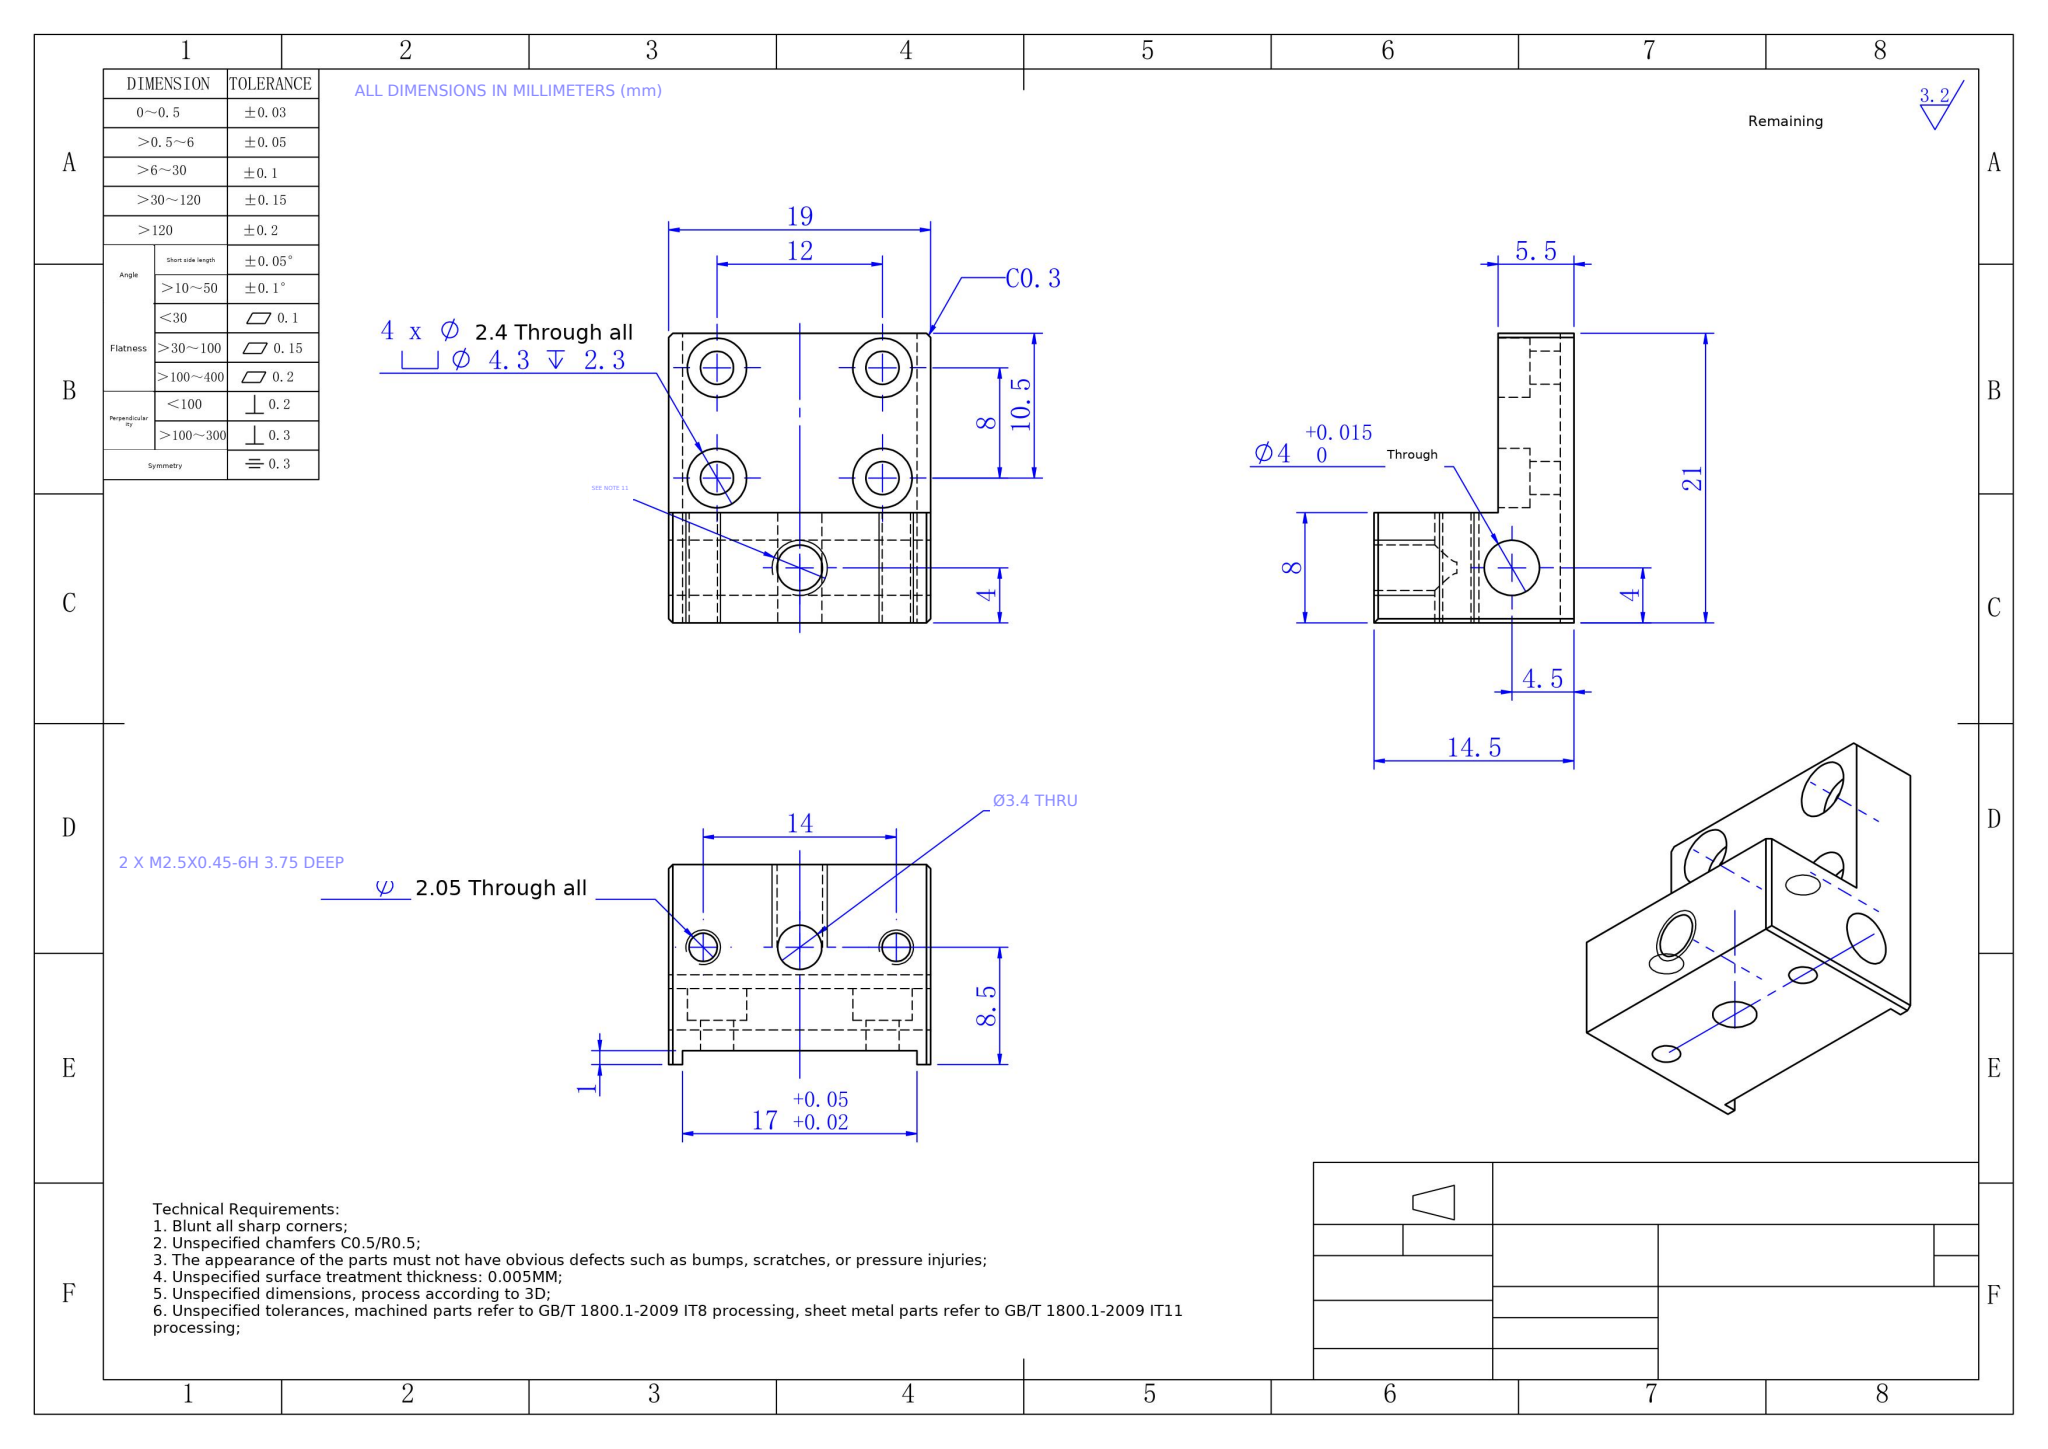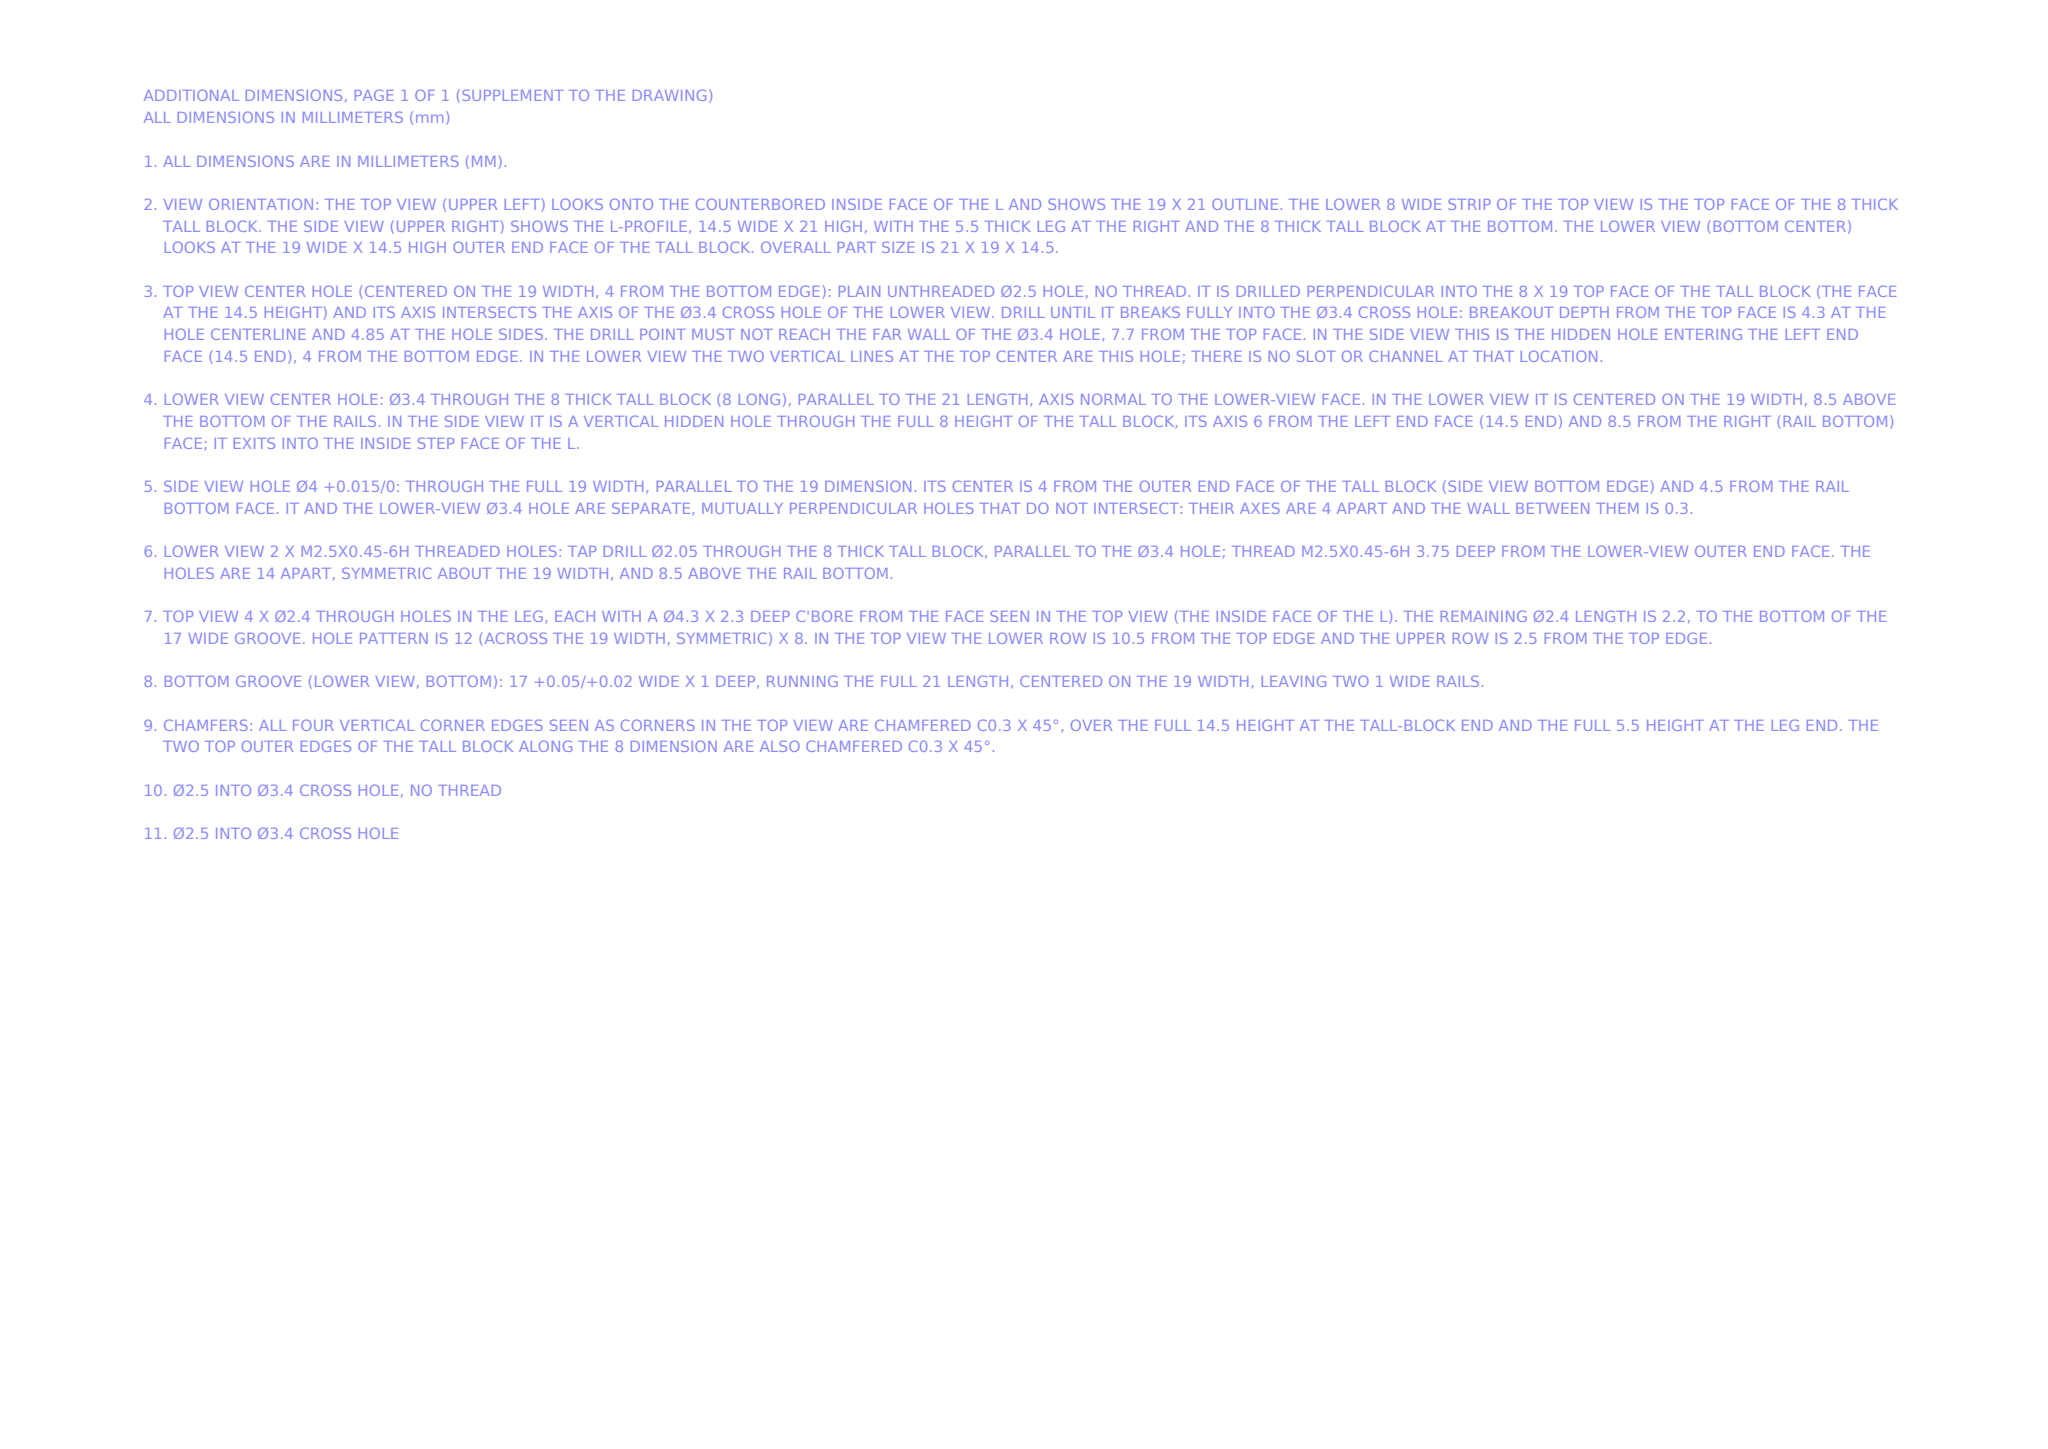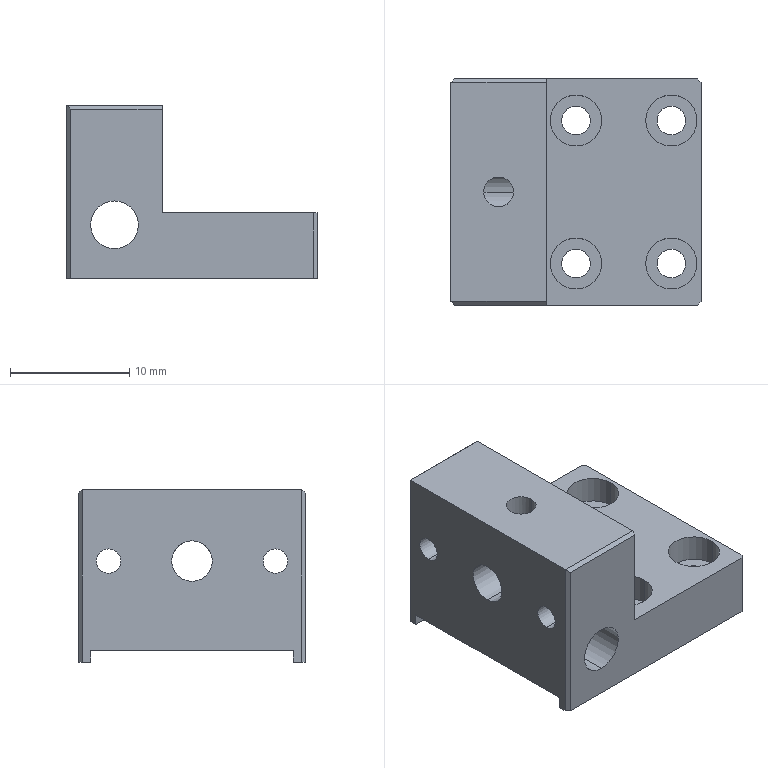Part | NX | mm | 1 solid | 48 faces | box 21 x 19 x 14.5 mm | volume 2644 mm3 | cylinder 26 | plane 22 | commonest cylinder face diameters 4.3 x8 2.4 x8 2.05 x4 2.5 x2 3.4 x2 4 x2